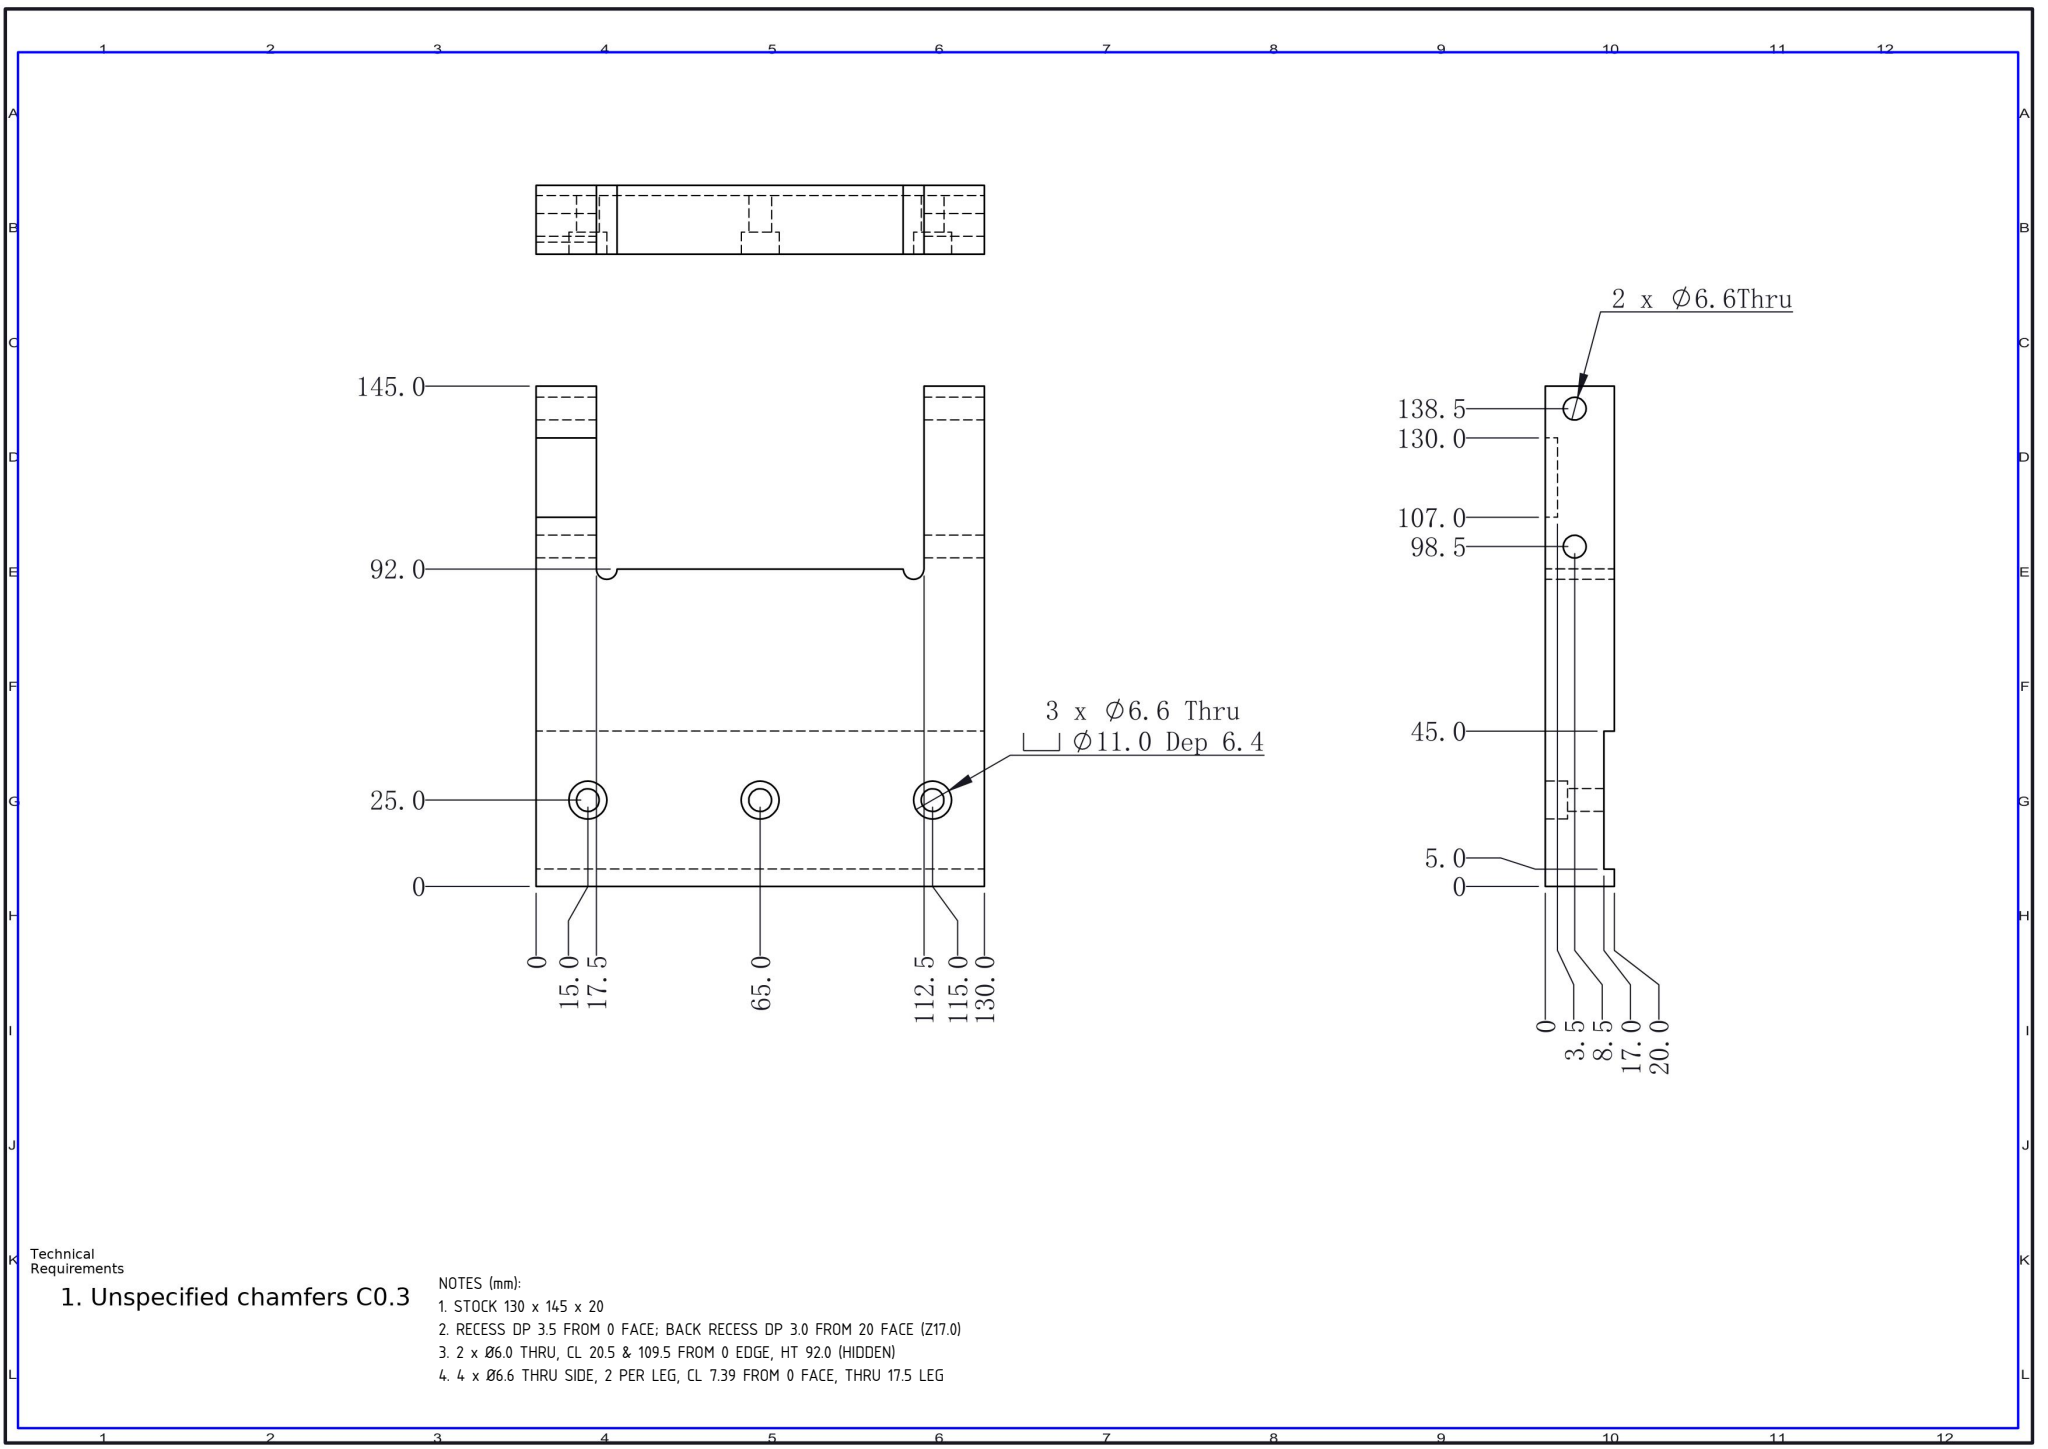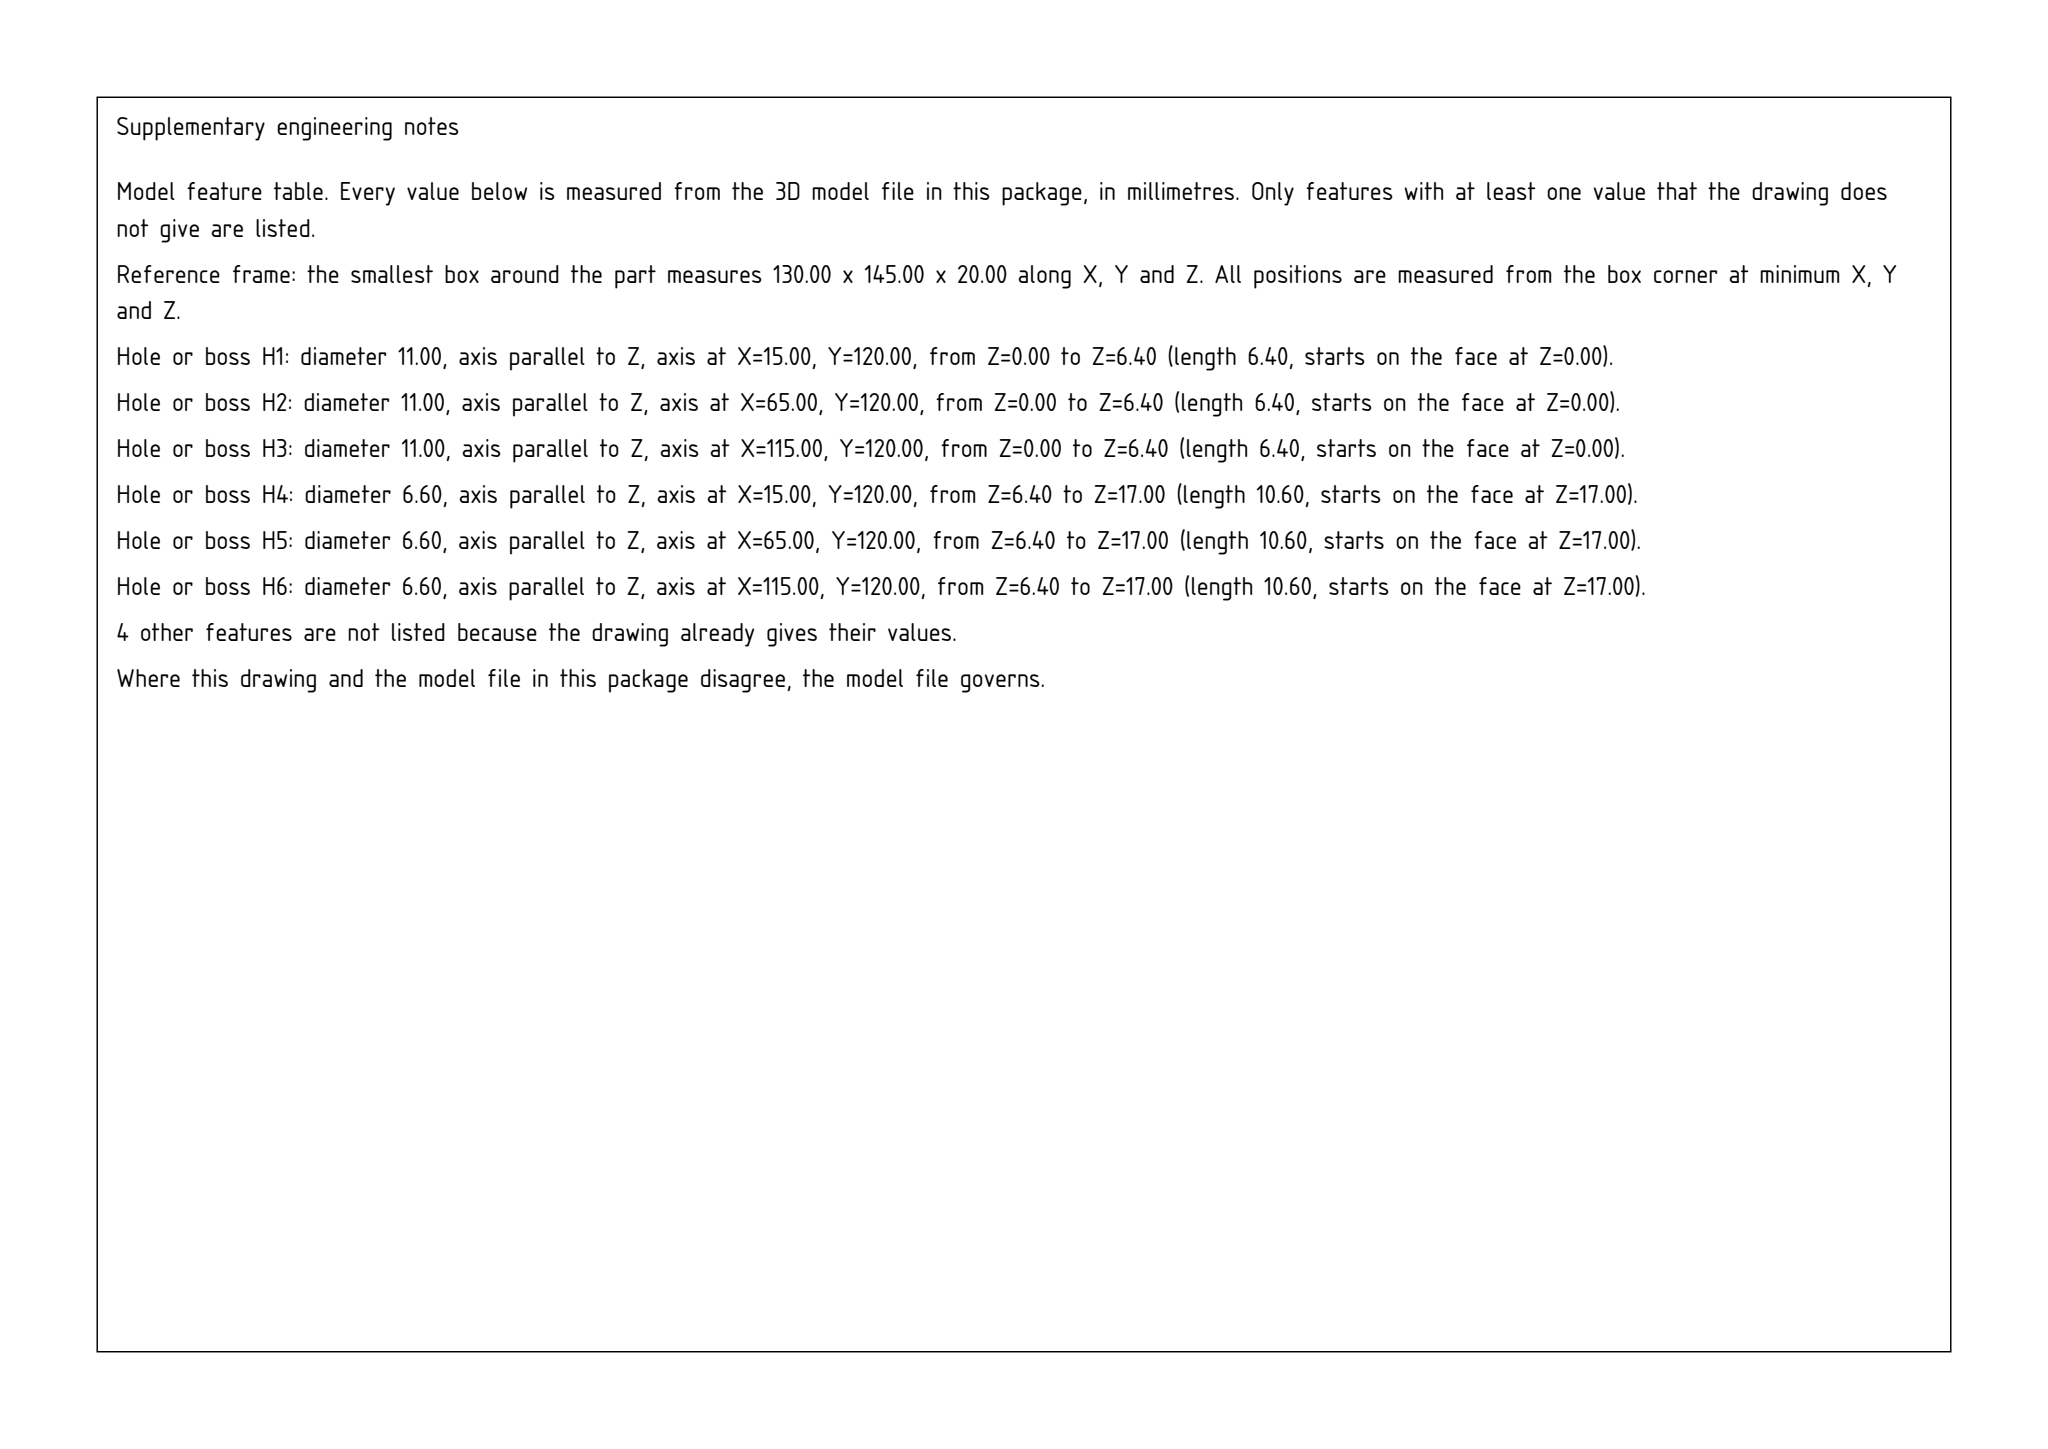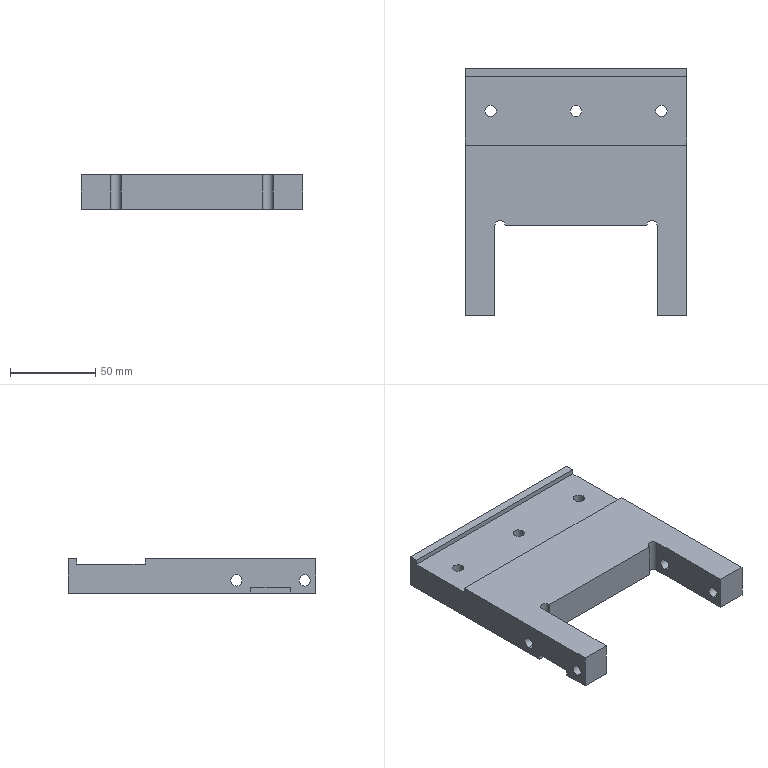Part | SolidWorks | mm | 1 solid | 43 faces | box 130 x 145 x 20 mm | volume 253418 mm3 | cylinder 22 | plane 21 | commonest cylinder face diameters 6.6 x14 11 x6 6 x2
Drawing notes:
STOCK 130 x 145 x 20 | from the solid: bbox_xyz 130.0 x 145.0 x 20.0
RECESS DP 3.5 FROM 0 FACE; BACK RECESS DP 3.0 FROM 20 FACE (Z17.0) | from the solid: z planes 0, 3.5, 17.0, 20.0; steps at y 100/38/15 = hts 45.0/107.0/130.0
2 x Ø6.0 THRU, CL 20.5 & 109.5 FROM 0 EDGE, HT 92.0 (HIDDEN) | from the solid: cylinders Ø6.0 axis z at (20.5,53) and (109.5,53), len 20 = full thk; 145-53=92.0
4 x Ø6.6 THRU SIDE, 2 PER LEG, CL 7.39 FROM 0 FACE, THRU 17.5 LEG | from the solid: cylinders Ø6.6 axis x at y=6.5 & 46.5, z=7.39, len 17.5, count 4; legs x 0-17.5 & 112.5-130
build123d program:
from build123d import *

# Parameters (mm, degrees)
SKETCH1_W                                       = 130
SKETCH1_H                                       = 145
BOSS_EXTRUDE1_DEPTH                             = 20
SKETCH2_W                                       = 130
SKETCH2_H                                       = 40
CUT_EXTRUDE1_DEPTH                              = 3
M6_HEX_SOCKET_HEAD_CAP_SCREW_CBORE1_D           = 6.6
M6_HEX_SOCKET_HEAD_CAP_SCREW_CBORE1_CBORE_D     = 11
M6_HEX_SOCKET_HEAD_CAP_SCREW_CBORE1_CBORE_DEPTH = 6.4
SKETCH8_W                                       = 95
SKETCH8_H                                       = 53
CUT_EXTRUDE2_DEPTH                              = 196.768
M6_CLEARANCE_HOLE1_D                            = 6.6
CUT_EXTRUDE3_REACH                              = 197.768
SKETCH11_W                                      = 3.5
SKETCH11_H                                      = 23
SKETCH12_R                                      = 3
CUT_EXTRUDE4_DEPTH                              = 196.768


with BuildPart() as part:
    # Sketch1 → Boss-Extrude1 (new body)
    with BuildSketch(Plane.XY):
        with Locations((65, -72.5)):
            Rectangle(SKETCH1_W, SKETCH1_H)
    extrude(amount=BOSS_EXTRUDE1_DEPTH)

    # Sketch2 → Cut-Extrude1 (cut)
    with BuildSketch(Plane.XY.offset(20)):
        with Locations((65, -25)):
            Rectangle(SKETCH2_W, SKETCH2_H)
    extrude(amount=-CUT_EXTRUDE1_DEPTH, mode=Mode.SUBTRACT)

    # M6 Hex Socket Head Cap Screw CBORE1 (through all)
    with Locations(Plane(origin=(0, 0, 0), x_dir=(-1, 0, 0), z_dir=(0, 0, -1))):
        with Locations((-15, -25), (-65, -25), (-115, -25)):
            CounterBoreHole(M6_HEX_SOCKET_HEAD_CAP_SCREW_CBORE1_D / 2, M6_HEX_SOCKET_HEAD_CAP_SCREW_CBORE1_CBORE_D / 2, M6_HEX_SOCKET_HEAD_CAP_SCREW_CBORE1_CBORE_DEPTH)

    # Sketch8 → Cut-Extrude2 (cut, through all)
    with BuildSketch(Plane(origin=(0, 0, 0), x_dir=(-1, 0, 0), z_dir=(0, 0, -1))):
        with Locations((-65, -118.5)):
            Rectangle(SKETCH8_W, SKETCH8_H)
    extrude(amount=-CUT_EXTRUDE2_DEPTH, mode=Mode.SUBTRACT)

    # M6 Clearance Hole1 (through all)
    with Locations(Plane.ZY):
        with Locations((7.393, -98.5), (7.393, -138.5)):
            Hole(M6_CLEARANCE_HOLE1_D / 2)

    # Sketch11 → Cut-Extrude3 (cut, up to next)
    with BuildSketch(Plane.ZY, mode=Mode.PRIVATE) as cut_extrude3_sk1:
        with Locations((1.75, -118.5)):
            Rectangle(SKETCH11_W, SKETCH11_H)
    cut_extrude3_tool1 = extrude(cut_extrude3_sk1.sketch, amount=-CUT_EXTRUDE3_REACH, mode=Mode.PRIVATE) & part.part
    add(cut_extrude3_tool1.solids().sort_by_distance((0, -118.5, 1.75))[0], mode=Mode.SUBTRACT)

    # Sketch12 → Cut-Extrude4 (cut, through all)
    with BuildSketch(Plane(origin=(0, 0, 0), x_dir=(-1, 0, 0), z_dir=(0, 0, -1))):
        with Locations((-20.5, -92)):
            Circle(SKETCH12_R)
        with Locations((-109.5, -92)):
            Circle(SKETCH12_R)
    extrude(amount=-CUT_EXTRUDE4_DEPTH, mode=Mode.SUBTRACT)


solid = part.part